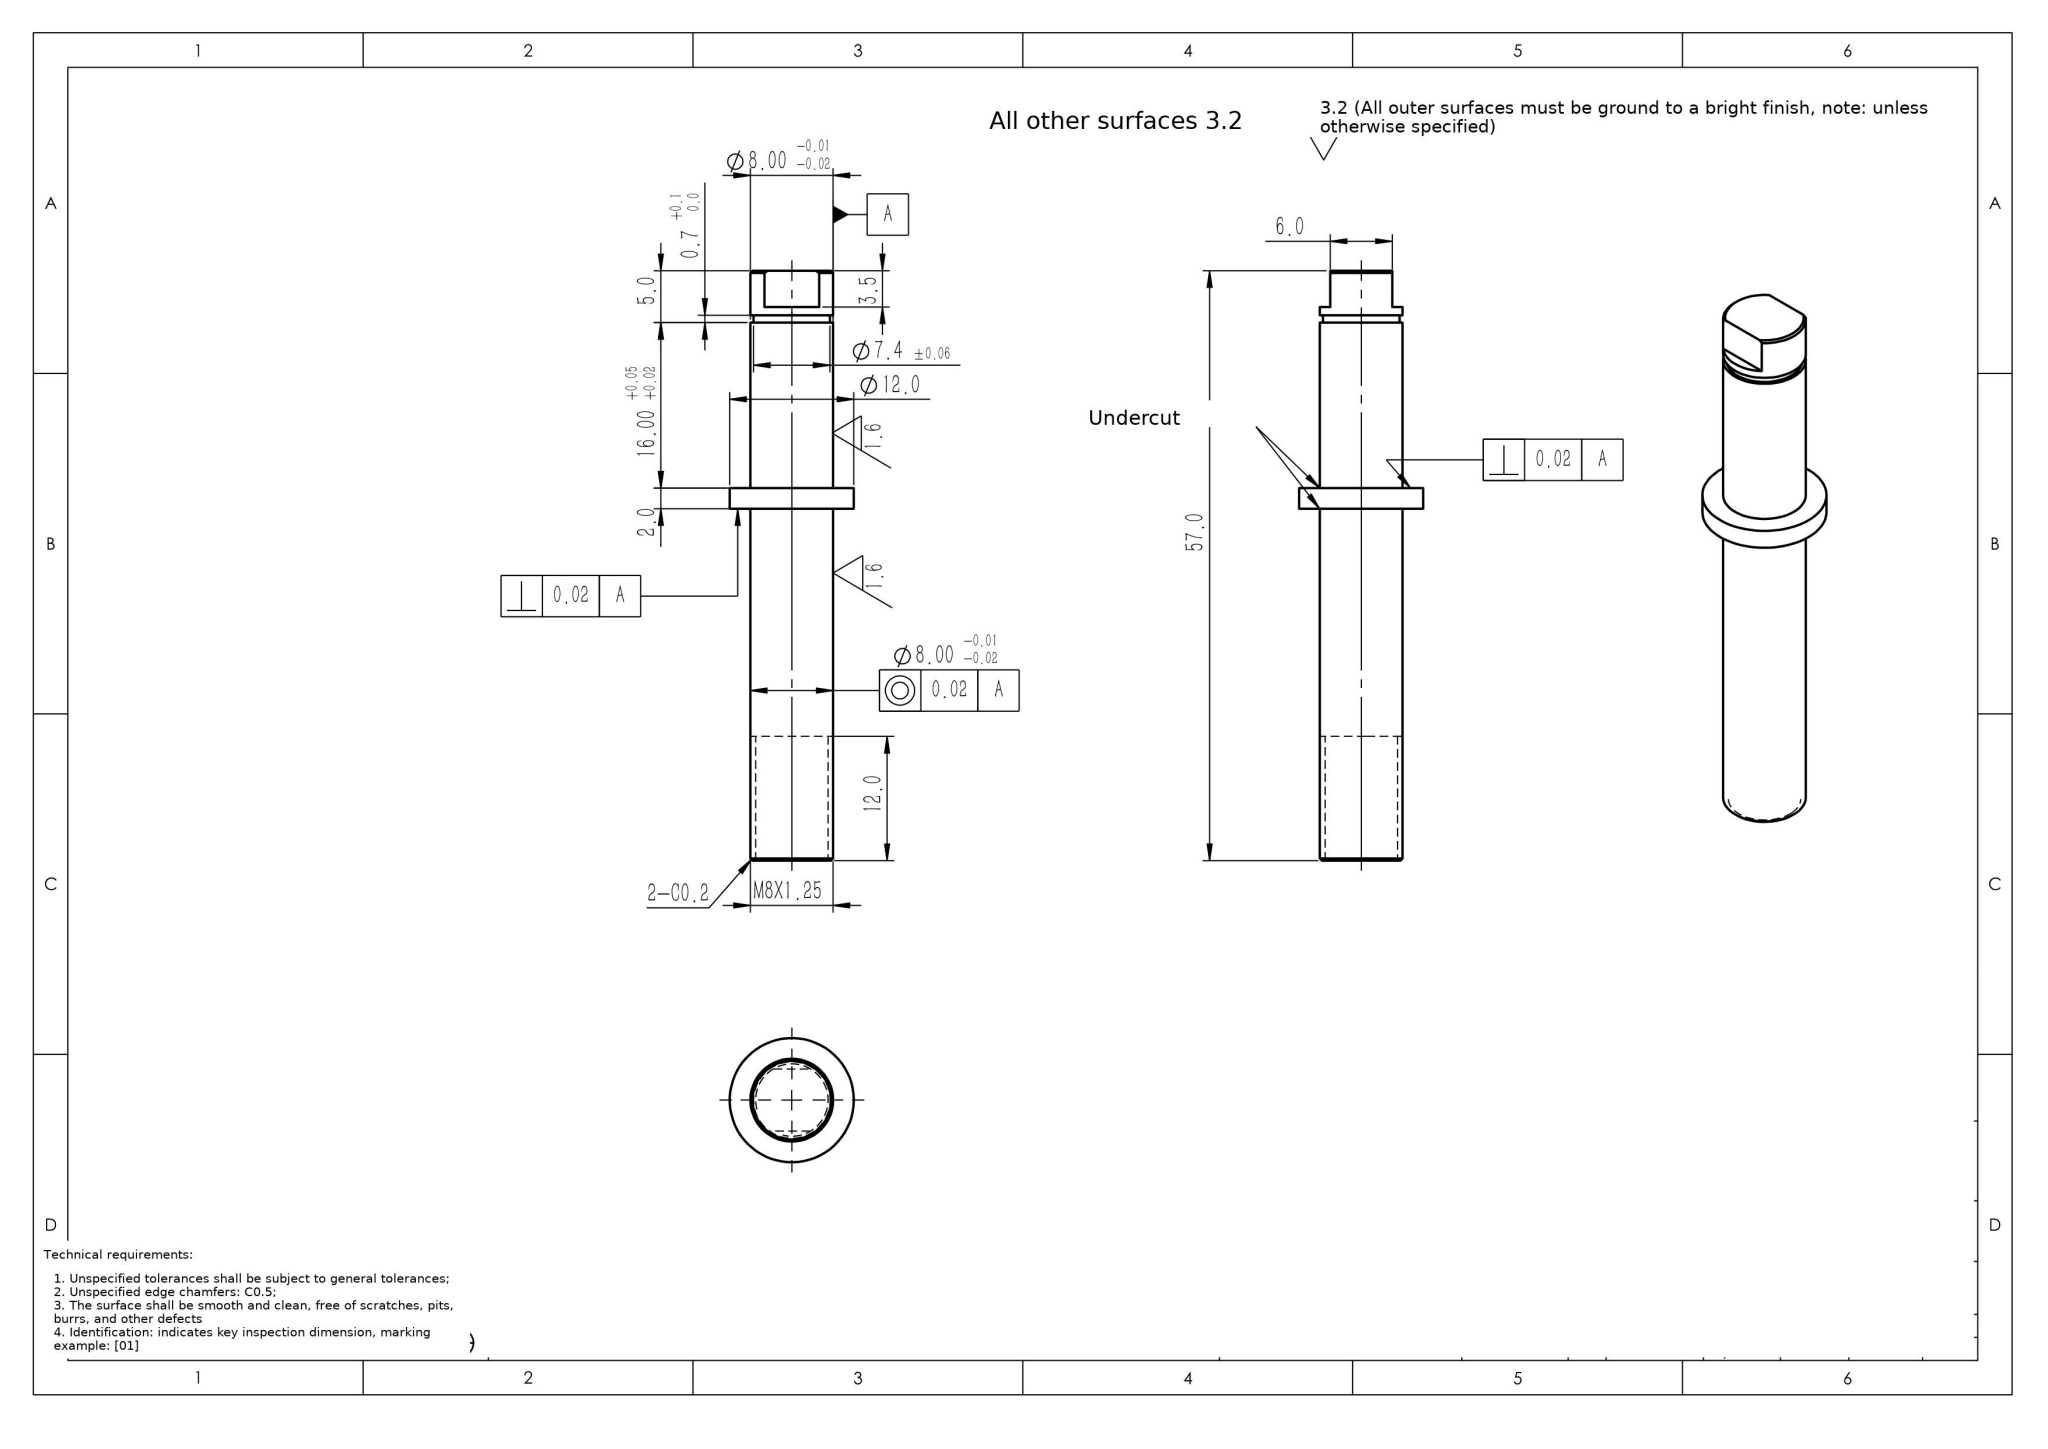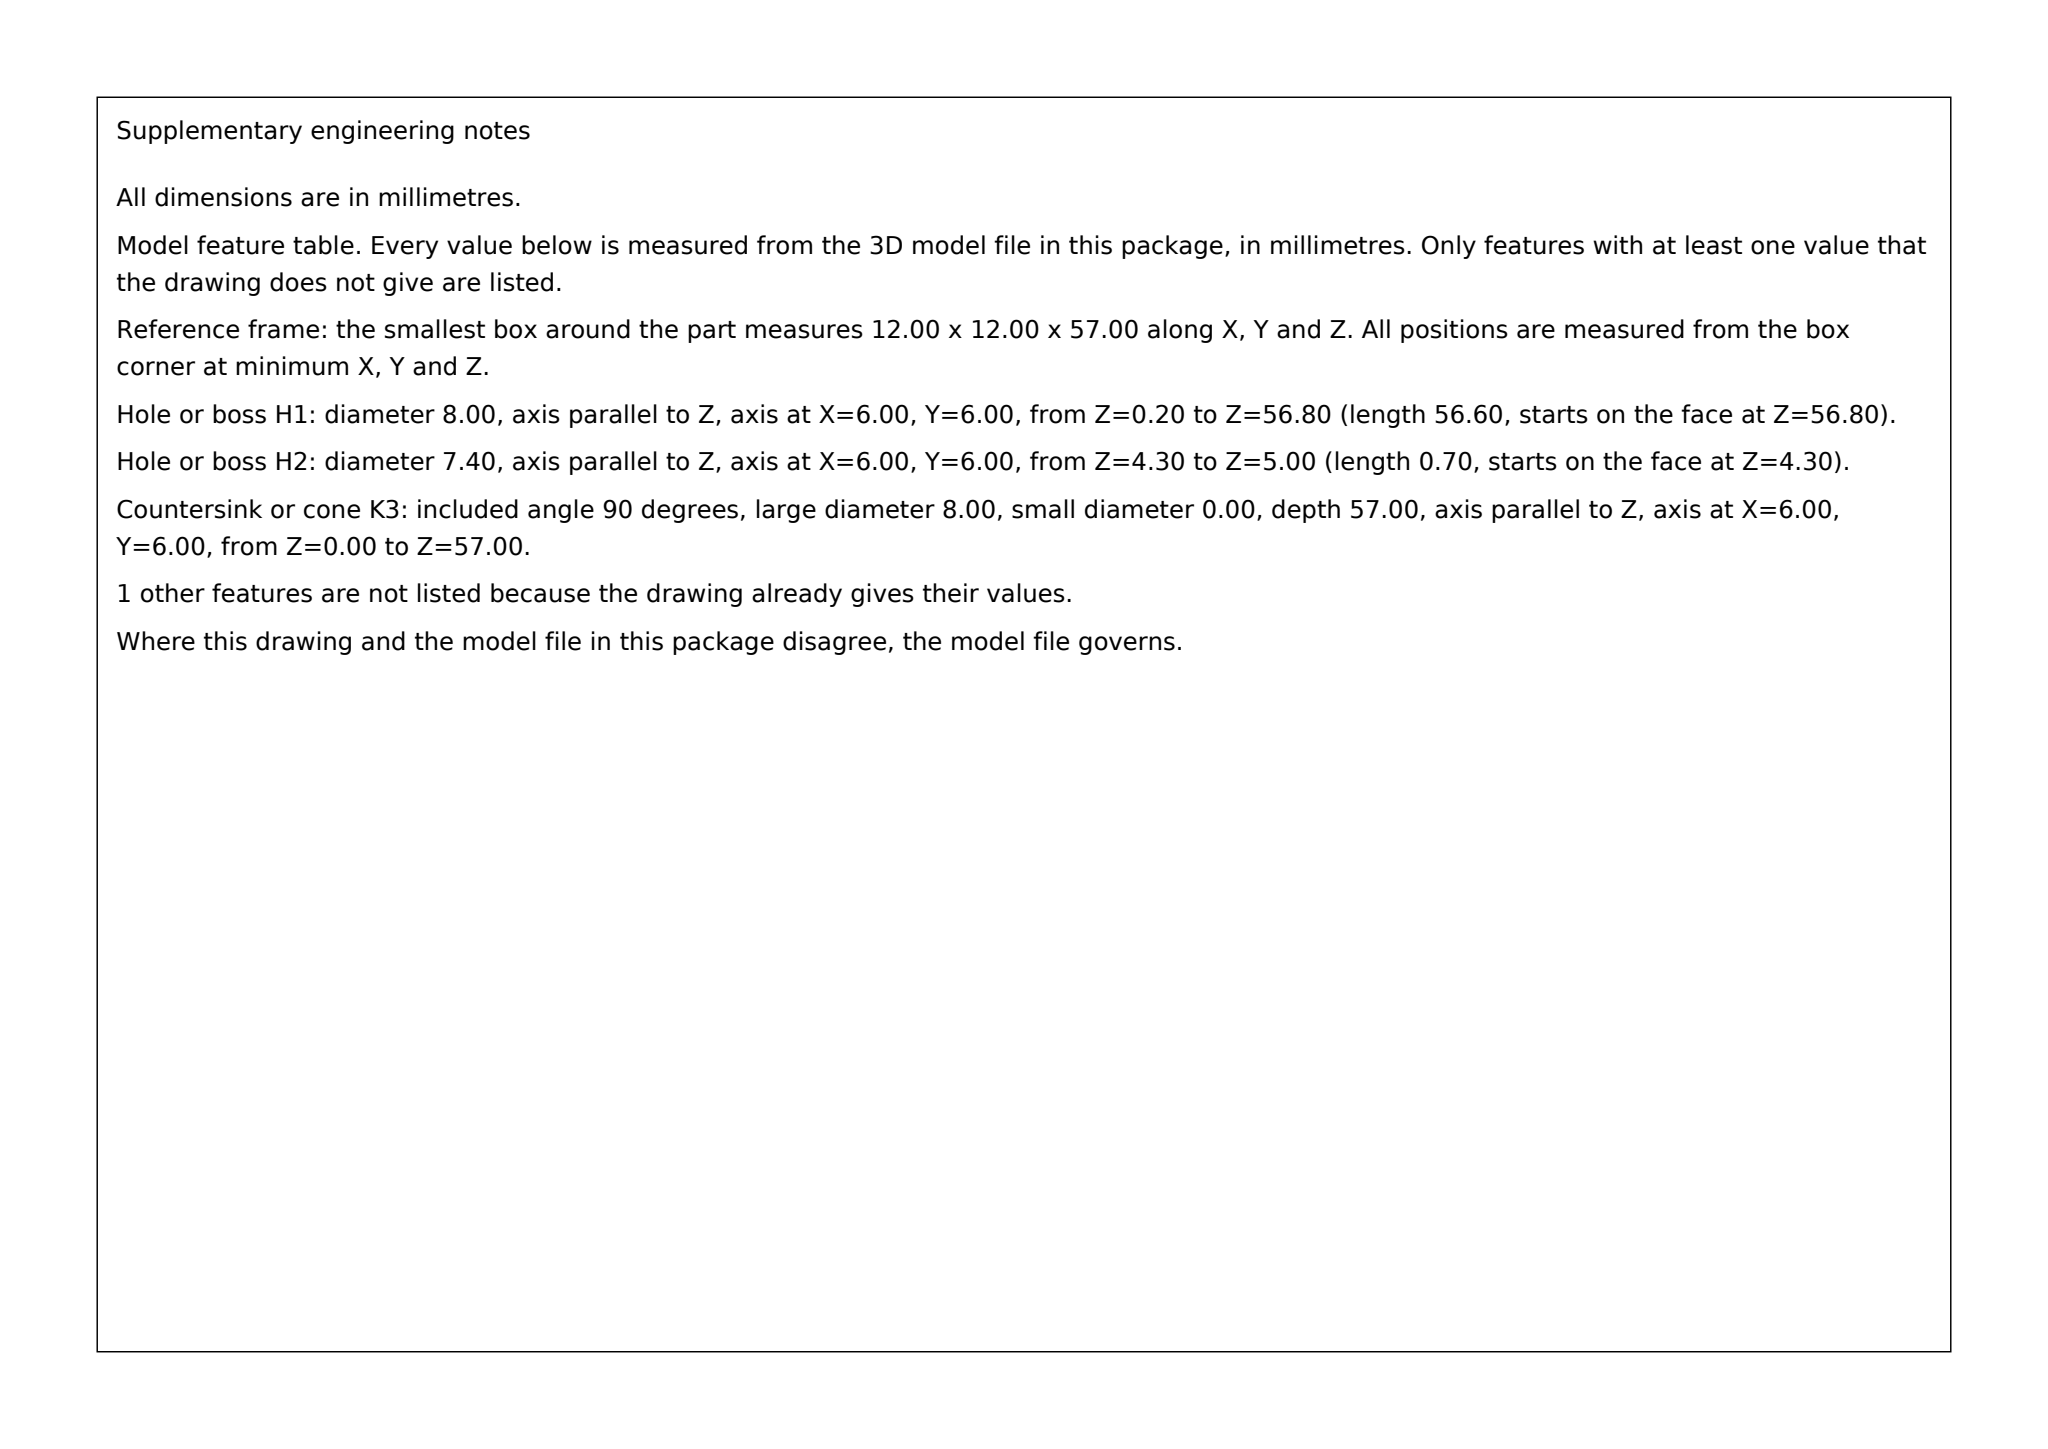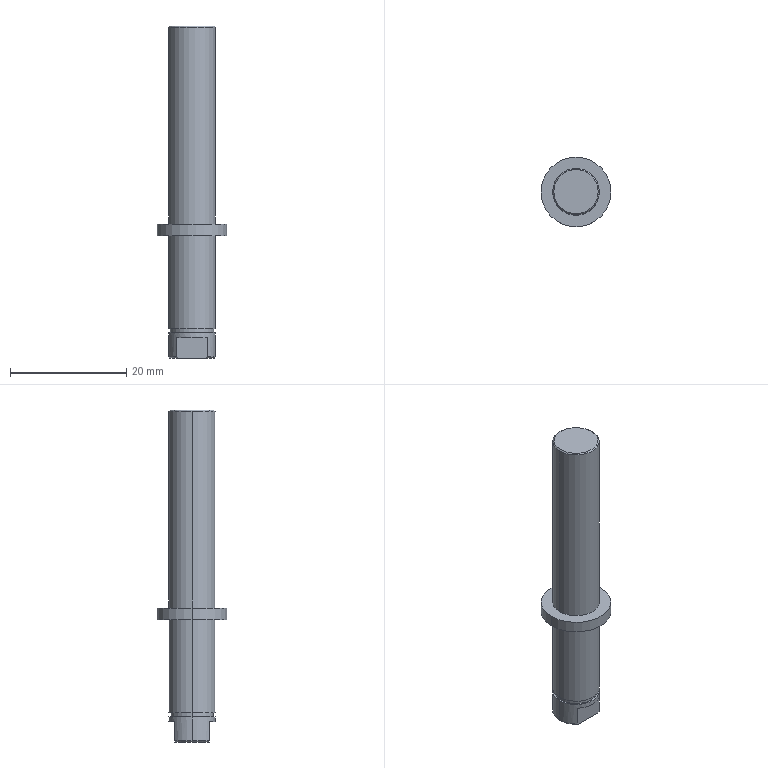Part | SolidWorks | mm | 1 solid | 25 faces | box 12 x 12 x 57 mm | volume 2960 mm3 | cylinder 10 | plane 10 | cone 5 | commonest cylinder face diameters 8 x6 7.4 x2 12 x2
build123d program:
from build123d import *

# Parameters (mm, degrees)
SKETCH1_R           = 6
BOSS_EXTRUDE1_DEPTH = 2
SKETCH2_R           = 4
BOSS_EXTRUDE2_DEPTH = 36
BOSS_EXTRUDE4_START = 21
SKETCH3_R           = 4
BOSS_EXTRUDE4_DEPTH = 21
SKETCH5_W           = 0.3
SKETCH5_H           = 0.7
CUT_EXTRUDE1_DEPTH  = 3.5
CHAMFER1_SIZE       = 0.2


with BuildPart() as part:
    # Sketch1 → Boss-Extrude1 (new body)
    with BuildSketch(Plane.XY):
        Circle(SKETCH1_R)
    extrude(amount=BOSS_EXTRUDE1_DEPTH)

    # Sketch2 → Boss-Extrude2 (add)
    with BuildSketch(Plane.XY):
        Circle(SKETCH2_R)
    extrude(amount=BOSS_EXTRUDE2_DEPTH)

    # Sketch3 → Boss-Extrude4 (add)
    with BuildSketch(Plane(origin=(0, 0, 0), x_dir=(-1, 0, 0), z_dir=(0, 0, -1)).offset(BOSS_EXTRUDE4_START)):
        with Locations(Location((0, 0, 0), (0, 0, 180))):
            Circle(SKETCH3_R)
    extrude(amount=-BOSS_EXTRUDE4_DEPTH)

    # Sketch5 → Cut-Revolve1 (revolve, cut)
    with BuildSketch(Plane(origin=(0, 0, 0), x_dir=(1, 0, 0), z_dir=(0, 1, 0))):
        with Locations((3.85, 16.35)):
            Rectangle(SKETCH5_W, SKETCH5_H)
    revolve(axis=Axis((0, 0, 0), (0, 0, -1)), mode=Mode.SUBTRACT)

    # Sketch6 → Cut-Extrude1 (cut)
    with BuildSketch(Plane(origin=(0, 0, -21), x_dir=(-1, 0, 0), z_dir=(0, 0, -1))):
        with BuildLine():
            Line((-2.646, 3), (2.646, 3))
            ThreePointArc((2.646, 3), (0, 4), (-2.646, 3))
        make_face()
        with BuildLine():
            Line((2.646, -3), (-2.646, -3))
            ThreePointArc((-2.646, -3), (0, -4), (2.646, -3))
        make_face()
    extrude(amount=-CUT_EXTRUDE1_DEPTH, mode=Mode.SUBTRACT)

    # Chamfer1
    chamfer1_edges = [part.edges().sort_by_distance(p)[0] for p in [
        (-4, 0, -21),
        (3.646, -1.646, -21),
        (-4, 0, 36),
    ]]
    chamfer(chamfer1_edges, length=CHAMFER1_SIZE)


solid = part.part
STEP:
#1=CARTESIAN_POINT('',(3.8,0.,36.));
#2=VERTEX_POINT('',#1);
#3=CARTESIAN_POINT('',(-3.8,0.,36.));
#4=VERTEX_POINT('',#3);
#5=CARTESIAN_POINT('',(0.,0.,36.));
#6=DIRECTION('',(0.,0.,1.));
#7=DIRECTION('',(1.,0.,0.));
#8=AXIS2_PLACEMENT_3D('',#5,#6,#7);
#9=CIRCLE('',#8,3.8);
#10=EDGE_CURVE('',#2,#4,#9,.T.);
#11=ORIENTED_EDGE('',*,*,#10,.F.);
#12=CARTESIAN_POINT('',(4.,0.,35.8));
#13=VERTEX_POINT('',#12);
#14=CARTESIAN_POINT('',(3.8,0.,36.));
#15=DIRECTION('',(0.7071,0.,-0.7071));
#16=VECTOR('',#15,1000.);
#17=LINE('',#14,#16);
#18=EDGE_CURVE('',#2,#13,#17,.T.);
#19=ORIENTED_EDGE('',*,*,#18,.T.);
#20=CARTESIAN_POINT('',(-4.,0.,35.8));
#21=VERTEX_POINT('',#20);
#22=CARTESIAN_POINT('',(0.,0.,35.8));
#23=DIRECTION('',(0.,0.,-1.));
#24=DIRECTION('',(1.,0.,0.));
#25=AXIS2_PLACEMENT_3D('',#22,#23,#24);
#26=CIRCLE('',#25,4.);
#27=EDGE_CURVE('',#21,#13,#26,.T.);
#28=ORIENTED_EDGE('',*,*,#27,.F.);
#29=CARTESIAN_POINT('',(-3.8,0.,36.));
#30=DIRECTION('',(-0.7071,0.,-0.7071));
#31=VECTOR('',#30,1000.);
#32=LINE('',#29,#31);
#33=EDGE_CURVE('',#4,#21,#32,.T.);
#34=ORIENTED_EDGE('',*,*,#33,.F.);
#35=EDGE_LOOP('',(#11,#19,#28,#34));
#36=FACE_OUTER_BOUND('',#35,.T.);
#37=CARTESIAN_POINT('',(0.,0.,36.));
#38=DIRECTION('',(0.,0.,-1.));
#39=DIRECTION('',(-1.,0.,0.));
#40=AXIS2_PLACEMENT_3D('',#37,#38,#39);
#41=CONICAL_SURFACE('',#40,3.8,0.7854);
#42=ADVANCED_FACE('',(#36),#41,.T.);
#43=CARTESIAN_POINT('',(3.8,0.,-21.));
#44=VERTEX_POINT('',#43);
#45=CARTESIAN_POINT('',(2.332,-3.,-21.));
#46=VERTEX_POINT('',#45);
#47=CARTESIAN_POINT('',(0.,0.,-21.));
#48=DIRECTION('',(0.,0.,-1.));
#49=DIRECTION('',(-1.,0.,0.));
#50=AXIS2_PLACEMENT_3D('',#47,#48,#49);
#51=CIRCLE('',#50,3.8);
#52=EDGE_CURVE('',#44,#46,#51,.T.);
#53=ORIENTED_EDGE('',*,*,#52,.F.);
#54=CARTESIAN_POINT('',(4.,0.,-20.8));
#55=VERTEX_POINT('',#54);
#56=CARTESIAN_POINT('',(3.8,0.,-21.));
#57=DIRECTION('',(0.7071,0.,0.7071));
#58=VECTOR('',#57,1000.);
#59=LINE('',#56,#58);
#60=EDGE_CURVE('',#44,#55,#59,.T.);
#61=ORIENTED_EDGE('',*,*,#60,.T.);
#62=CARTESIAN_POINT('',(2.646,-3.,-20.8));
#63=VERTEX_POINT('',#62);
#64=CARTESIAN_POINT('',(0.,0.,-20.8));
#65=DIRECTION('',(0.,0.,1.));
#66=DIRECTION('',(-1.,0.,0.));
#67=AXIS2_PLACEMENT_3D('',#64,#65,#66);
#68=CIRCLE('',#67,4.);
#69=EDGE_CURVE('',#63,#55,#68,.T.);
#70=ORIENTED_EDGE('',*,*,#69,.F.);
#71=CARTESIAN_POINT('',(2.332,-3.,-21.));
#72=CARTESIAN_POINT('',(2.438,-3.,-20.935));
#73=CARTESIAN_POINT('',(2.542,-3.,-20.868));
#74=CARTESIAN_POINT('',(2.646,-3.,-20.8));
#75=B_SPLINE_CURVE_WITH_KNOTS('',3,(#71,#72,#73,#74),.UNSPECIFIED.,.F.,.F.,(4,4),(0.,0.0003718),.UNSPECIFIED.);
#76=EDGE_CURVE('',#46,#63,#75,.T.);
#77=ORIENTED_EDGE('',*,*,#76,.F.);
#78=EDGE_LOOP('',(#53,#61,#70,#77));
#79=FACE_OUTER_BOUND('',#78,.T.);
#80=CARTESIAN_POINT('',(0.,0.,-21.));
#81=DIRECTION('',(0.,0.,1.));
#82=DIRECTION('',(1.,0.,0.));
#83=AXIS2_PLACEMENT_3D('',#80,#81,#82);
#84=CONICAL_SURFACE('',#83,3.8,0.7854);
#85=ADVANCED_FACE('',(#79),#84,.T.);
#86=CARTESIAN_POINT('',(-2.646,3.,-20.8));
#87=VERTEX_POINT('',#86);
#88=CARTESIAN_POINT('',(-4.,0.,-20.8));
#89=VERTEX_POINT('',#88);
#90=CARTESIAN_POINT('',(0.,0.,-20.8));
#91=DIRECTION('',(0.,0.,1.));
#92=DIRECTION('',(-1.,-0.,0.));
#93=AXIS2_PLACEMENT_3D('',#90,#91,#92);
#94=CIRCLE('',#93,4.);
#95=EDGE_CURVE('',#87,#89,#94,.T.);
#96=ORIENTED_EDGE('',*,*,#95,.T.);
#97=CARTESIAN_POINT('',(-4.,0.,-16.7));
#98=VERTEX_POINT('',#97);
#99=CARTESIAN_POINT('',(-4.,0.,-21.));
#100=DIRECTION('',(0.,0.,1.));
#101=VECTOR('',#100,1000.);
#102=LINE('',#99,#101);
#103=EDGE_CURVE('',#89,#98,#102,.T.);
#104=ORIENTED_EDGE('',*,*,#103,.T.);
#105=CARTESIAN_POINT('',(4.,0.,-16.7));
#106=VERTEX_POINT('',#105);
#107=CARTESIAN_POINT('',(0.,0.,-16.7));
#108=DIRECTION('',(0.,0.,1.));
#109=DIRECTION('',(1.,0.,0.));
#110=AXIS2_PLACEMENT_3D('',#107,#108,#109);
#111=CIRCLE('',#110,4.);
#112=EDGE_CURVE('',#106,#98,#111,.T.);
#113=ORIENTED_EDGE('',*,*,#112,.F.);
#114=CARTESIAN_POINT('',(4.,0.,-21.));
#115=DIRECTION('',(0.,0.,1.));
#116=VECTOR('',#115,1000.);
#117=LINE('',#114,#116);
#118=EDGE_CURVE('',#55,#106,#117,.T.);
#119=ORIENTED_EDGE('',*,*,#118,.F.);
#120=CARTESIAN_POINT('',(2.646,3.,-20.8));
#121=VERTEX_POINT('',#120);
#122=CARTESIAN_POINT('',(0.,0.,-20.8));
#123=DIRECTION('',(0.,0.,1.));
#124=DIRECTION('',(-1.,0.,0.));
#125=AXIS2_PLACEMENT_3D('',#122,#123,#124);
#126=CIRCLE('',#125,4.);
#127=EDGE_CURVE('',#55,#121,#126,.T.);
#128=ORIENTED_EDGE('',*,*,#127,.T.);
#129=CARTESIAN_POINT('',(2.646,3.,-17.5));
#130=VERTEX_POINT('',#129);
#131=CARTESIAN_POINT('',(2.646,3.,-17.5));
#132=DIRECTION('',(0.,0.,-1.));
#133=VECTOR('',#132,1000.);
#134=LINE('',#131,#133);
#135=EDGE_CURVE('',#130,#121,#134,.T.);
#136=ORIENTED_EDGE('',*,*,#135,.F.);
#137=CARTESIAN_POINT('',(-2.646,3.,-17.5));
#138=VERTEX_POINT('',#137);
#139=CARTESIAN_POINT('',(0.,0.,-17.5));
#140=DIRECTION('',(0.,0.,-1.));
#141=DIRECTION('',(-1.,0.,0.));
#142=AXIS2_PLACEMENT_3D('',#139,#140,#141);
#143=CIRCLE('',#142,4.);
#144=EDGE_CURVE('',#138,#130,#143,.T.);
#145=ORIENTED_EDGE('',*,*,#144,.F.);
#146=CARTESIAN_POINT('',(-2.646,3.,-17.5));
#147=DIRECTION('',(0.,0.,-1.));
#148=VECTOR('',#147,1000.);
#149=LINE('',#146,#148);
#150=EDGE_CURVE('',#138,#87,#149,.T.);
#151=ORIENTED_EDGE('',*,*,#150,.T.);
#152=EDGE_LOOP('',(#96,#104,#113,#119,#128,#136,#145,#151));
#153=FACE_OUTER_BOUND('',#152,.T.);
#154=CARTESIAN_POINT('',(0.,0.,-21.));
#155=DIRECTION('',(0.,0.,1.));
#156=DIRECTION('',(1.,0.,0.));
#157=AXIS2_PLACEMENT_3D('',#154,#155,#156);
#158=CYLINDRICAL_SURFACE('',#157,4.);
#159=ADVANCED_FACE('',(#153),#158,.T.);
#160=CARTESIAN_POINT('',(3.7,0.,-16.7));
#161=VERTEX_POINT('',#160);
#162=CARTESIAN_POINT('',(-3.7,0.,-16.7));
#163=VERTEX_POINT('',#162);
#164=CARTESIAN_POINT('',(0.,0.,-16.7));
#165=DIRECTION('',(0.,0.,1.));
#166=DIRECTION('',(1.,0.,0.));
#167=AXIS2_PLACEMENT_3D('',#164,#165,#166);
#168=CIRCLE('',#167,3.7);
#169=EDGE_CURVE('',#161,#163,#168,.T.);
#170=ORIENTED_EDGE('',*,*,#169,.T.);
#171=CARTESIAN_POINT('',(-3.7,0.,-16.));
#172=VERTEX_POINT('',#171);
#173=CARTESIAN_POINT('',(-3.7,0.,0.));
#174=DIRECTION('',(0.,0.,1.));
#175=VECTOR('',#174,1000.);
#176=LINE('',#173,#175);
#177=EDGE_CURVE('',#163,#172,#176,.T.);
#178=ORIENTED_EDGE('',*,*,#177,.T.);
#179=CARTESIAN_POINT('',(3.7,0.,-16.));
#180=VERTEX_POINT('',#179);
#181=CARTESIAN_POINT('',(0.,0.,-16.));
#182=DIRECTION('',(0.,0.,1.));
#183=DIRECTION('',(1.,0.,0.));
#184=AXIS2_PLACEMENT_3D('',#181,#182,#183);
#185=CIRCLE('',#184,3.7);
#186=EDGE_CURVE('',#180,#172,#185,.T.);
#187=ORIENTED_EDGE('',*,*,#186,.F.);
#188=CARTESIAN_POINT('',(3.7,0.,0.));
#189=DIRECTION('',(0.,0.,1.));
#190=VECTOR('',#189,1000.);
#191=LINE('',#188,#190);
#192=EDGE_CURVE('',#161,#180,#191,.T.);
#193=ORIENTED_EDGE('',*,*,#192,.F.);
#194=EDGE_LOOP('',(#170,#178,#187,#193));
#195=FACE_OUTER_BOUND('',#194,.T.);
#196=CARTESIAN_POINT('',(0.,0.,0.));
#197=DIRECTION('',(0.,0.,1.));
#198=DIRECTION('',(1.,0.,0.));
#199=AXIS2_PLACEMENT_3D('',#196,#197,#198);
#200=CYLINDRICAL_SURFACE('',#199,3.7);
#201=ADVANCED_FACE('',(#195),#200,.T.);
#202=ORIENTED_EDGE('',*,*,#27,.T.);
#203=CARTESIAN_POINT('',(4.,0.,2.));
#204=VERTEX_POINT('',#203);
#205=CARTESIAN_POINT('',(4.,0.,36.));
#206=DIRECTION('',(0.,0.,-1.));
#207=VECTOR('',#206,1000.);
#208=LINE('',#205,#207);
#209=EDGE_CURVE('',#13,#204,#208,.T.);
#210=ORIENTED_EDGE('',*,*,#209,.T.);
#211=CARTESIAN_POINT('',(-4.,0.,2.));
#212=VERTEX_POINT('',#211);
#213=CARTESIAN_POINT('',(0.,0.,2.));
#214=DIRECTION('',(0.,0.,-1.));
#215=DIRECTION('',(1.,0.,0.));
#216=AXIS2_PLACEMENT_3D('',#213,#214,#215);
#217=CIRCLE('',#216,4.);
#218=EDGE_CURVE('',#212,#204,#217,.T.);
#219=ORIENTED_EDGE('',*,*,#218,.F.);
#220=CARTESIAN_POINT('',(-4.,0.,36.));
#221=DIRECTION('',(0.,0.,-1.));
#222=VECTOR('',#221,1000.);
#223=LINE('',#220,#222);
#224=EDGE_CURVE('',#21,#212,#223,.T.);
#225=ORIENTED_EDGE('',*,*,#224,.F.);
#226=EDGE_LOOP('',(#202,#210,#219,#225));
#227=FACE_OUTER_BOUND('',#226,.T.);
#228=CARTESIAN_POINT('',(0.,0.,36.));
#229=DIRECTION('',(0.,0.,-1.));
#230=DIRECTION('',(-1.,0.,0.));
#231=AXIS2_PLACEMENT_3D('',#228,#229,#230);
#232=CYLINDRICAL_SURFACE('',#231,4.);
#233=ADVANCED_FACE('',(#227),#232,.T.);
#234=CARTESIAN_POINT('',(6.,0.,2.));
#235=VERTEX_POINT('',#234);
#236=CARTESIAN_POINT('',(-6.,0.,2.));
#237=VERTEX_POINT('',#236);
#238=CARTESIAN_POINT('',(0.,0.,2.));
#239=DIRECTION('',(0.,0.,1.));
#240=DIRECTION('',(1.,0.,0.));
#241=AXIS2_PLACEMENT_3D('',#238,#239,#240);
#242=CIRCLE('',#241,6.);
#243=EDGE_CURVE('',#235,#237,#242,.T.);
#244=ORIENTED_EDGE('',*,*,#243,.F.);
#245=CARTESIAN_POINT('',(6.,0.,0.));
#246=VERTEX_POINT('',#245);
#247=CARTESIAN_POINT('',(6.,0.,2.));
#248=DIRECTION('',(0.,0.,-1.));
#249=VECTOR('',#248,1000.);
#250=LINE('',#247,#249);
#251=EDGE_CURVE('',#235,#246,#250,.T.);
#252=ORIENTED_EDGE('',*,*,#251,.T.);
#253=CARTESIAN_POINT('',(-6.,0.,0.));
#254=VERTEX_POINT('',#253);
#255=CARTESIAN_POINT('',(0.,0.,0.));
#256=DIRECTION('',(0.,0.,1.));
#257=DIRECTION('',(1.,0.,0.));
#258=AXIS2_PLACEMENT_3D('',#255,#256,#257);
#259=CIRCLE('',#258,6.);
#260=EDGE_CURVE('',#246,#254,#259,.T.);
#261=ORIENTED_EDGE('',*,*,#260,.T.);
#262=CARTESIAN_POINT('',(-6.,0.,2.));
#263=DIRECTION('',(0.,0.,-1.));
#264=VECTOR('',#263,1000.);
#265=LINE('',#262,#264);
#266=EDGE_CURVE('',#237,#254,#265,.T.);
#267=ORIENTED_EDGE('',*,*,#266,.F.);
#268=EDGE_LOOP('',(#244,#252,#261,#267));
#269=FACE_OUTER_BOUND('',#268,.T.);
#270=CARTESIAN_POINT('',(0.,0.,2.));
#271=DIRECTION('',(0.,0.,-1.));
#272=DIRECTION('',(-1.,0.,0.));
#273=AXIS2_PLACEMENT_3D('',#270,#271,#272);
#274=CYLINDRICAL_SURFACE('',#273,6.);
#275=ADVANCED_FACE('',(#269),#274,.T.);
#276=CARTESIAN_POINT('',(4.,0.,-16.));
#277=VERTEX_POINT('',#276);
#278=CARTESIAN_POINT('',(-4.,0.,-16.));
#279=VERTEX_POINT('',#278);
#280=CARTESIAN_POINT('',(0.,0.,-16.));
#281=DIRECTION('',(0.,0.,1.));
#282=DIRECTION('',(1.,0.,0.));
#283=AXIS2_PLACEMENT_3D('',#280,#281,#282);
#284=CIRCLE('',#283,4.);
#285=EDGE_CURVE('',#277,#279,#284,.T.);
#286=ORIENTED_EDGE('',*,*,#285,.T.);
#287=CARTESIAN_POINT('',(-4.,0.,0.));
#288=VERTEX_POINT('',#287);
#289=CARTESIAN_POINT('',(-4.,0.,-21.));
#290=DIRECTION('',(0.,0.,1.));
#291=VECTOR('',#290,1000.);
#292=LINE('',#289,#291);
#293=EDGE_CURVE('',#279,#288,#292,.T.);
#294=ORIENTED_EDGE('',*,*,#293,.T.);
#295=CARTESIAN_POINT('',(4.,0.,0.));
#296=VERTEX_POINT('',#295);
#297=CARTESIAN_POINT('',(0.,0.,0.));
#298=DIRECTION('',(0.,0.,-1.));
#299=DIRECTION('',(1.,0.,0.));
#300=AXIS2_PLACEMENT_3D('',#297,#298,#299);
#301=CIRCLE('',#300,4.);
#302=EDGE_CURVE('',#288,#296,#301,.T.);
#303=ORIENTED_EDGE('',*,*,#302,.T.);
#304=CARTESIAN_POINT('',(4.,0.,-21.));
#305=DIRECTION('',(0.,0.,1.));
#306=VECTOR('',#305,1000.);
#307=LINE('',#304,#306);
#308=EDGE_CURVE('',#277,#296,#307,.T.);
#309=ORIENTED_EDGE('',*,*,#308,.F.);
#310=EDGE_LOOP('',(#286,#294,#303,#309));
#311=FACE_OUTER_BOUND('',#310,.T.);
#312=CARTESIAN_POINT('',(0.,0.,-21.));
#313=DIRECTION('',(0.,0.,1.));
#314=DIRECTION('',(1.,0.,0.));
#315=AXIS2_PLACEMENT_3D('',#312,#313,#314);
#316=CYLINDRICAL_SURFACE('',#315,4.);
#317=ADVANCED_FACE('',(#311),#316,.T.);
#318=ORIENTED_EDGE('',*,*,#293,.F.);
#319=CARTESIAN_POINT('',(0.,0.,-16.));
#320=DIRECTION('',(0.,0.,1.));
#321=DIRECTION('',(1.,0.,0.));
#322=AXIS2_PLACEMENT_3D('',#319,#320,#321);
#323=CIRCLE('',#322,4.);
#324=EDGE_CURVE('',#279,#277,#323,.T.);
#325=ORIENTED_EDGE('',*,*,#324,.T.);
#326=ORIENTED_EDGE('',*,*,#308,.T.);
#327=CARTESIAN_POINT('',(0.,0.,0.));
#328=DIRECTION('',(0.,0.,-1.));
#329=DIRECTION('',(1.,0.,0.));
#330=AXIS2_PLACEMENT_3D('',#327,#328,#329);
#331=CIRCLE('',#330,4.);
#332=EDGE_CURVE('',#296,#288,#331,.T.);
#333=ORIENTED_EDGE('',*,*,#332,.T.);
#334=EDGE_LOOP('',(#318,#325,#326,#333));
#335=FACE_OUTER_BOUND('',#334,.T.);
#336=CARTESIAN_POINT('',(0.,0.,-21.));
#337=DIRECTION('',(0.,0.,1.));
#338=DIRECTION('',(1.,0.,0.));
#339=AXIS2_PLACEMENT_3D('',#336,#337,#338);
#340=CYLINDRICAL_SURFACE('',#339,4.);
#341=ADVANCED_FACE('',(#335),#340,.T.);
#342=CARTESIAN_POINT('',(0.,0.,0.));
#343=DIRECTION('',(0.,0.,1.));
#344=DIRECTION('',(1.,0.,0.));
#345=AXIS2_PLACEMENT_3D('',#342,#343,#344);
#346=CIRCLE('',#345,6.);
#347=EDGE_CURVE('',#254,#246,#346,.T.);
#348=ORIENTED_EDGE('',*,*,#347,.F.);
#349=ORIENTED_EDGE('',*,*,#260,.F.);
#350=EDGE_LOOP('',(#348,#349));
#351=FACE_OUTER_BOUND('',#350,.T.);
#352=ORIENTED_EDGE('',*,*,#332,.F.);
#353=ORIENTED_EDGE('',*,*,#302,.F.);
#354=EDGE_LOOP('',(#352,#353));
#355=FACE_BOUND('',#354,.T.);
#356=CARTESIAN_POINT('',(0.,0.,0.));
#357=DIRECTION('',(0.,0.,1.));
#358=DIRECTION('',(1.,0.,0.));
#359=AXIS2_PLACEMENT_3D('',#356,#357,#358);
#360=PLANE('',#359);
#361=ADVANCED_FACE('',(#351,#355),#360,.F.);
#362=CARTESIAN_POINT('',(0.,0.,2.));
#363=DIRECTION('',(0.,0.,1.));
#364=DIRECTION('',(1.,0.,0.));
#365=AXIS2_PLACEMENT_3D('',#362,#363,#364);
#366=CIRCLE('',#365,6.);
#367=EDGE_CURVE('',#237,#235,#366,.T.);
#368=ORIENTED_EDGE('',*,*,#367,.T.);
#369=ORIENTED_EDGE('',*,*,#243,.T.);
#370=EDGE_LOOP('',(#368,#369));
#371=FACE_OUTER_BOUND('',#370,.T.);
#372=ORIENTED_EDGE('',*,*,#218,.T.);
#373=CARTESIAN_POINT('',(0.,0.,2.));
#374=DIRECTION('',(0.,0.,-1.));
#375=DIRECTION('',(1.,0.,0.));
#376=AXIS2_PLACEMENT_3D('',#373,#374,#375);
#377=CIRCLE('',#376,4.);
#378=EDGE_CURVE('',#204,#212,#377,.T.);
#379=ORIENTED_EDGE('',*,*,#378,.T.);
#380=EDGE_LOOP('',(#372,#379));
#381=FACE_BOUND('',#380,.T.);
#382=CARTESIAN_POINT('',(0.,0.,2.));
#383=DIRECTION('',(0.,0.,1.));
#384=DIRECTION('',(1.,0.,0.));
#385=AXIS2_PLACEMENT_3D('',#382,#383,#384);
#386=PLANE('',#385);
#387=ADVANCED_FACE('',(#371,#381),#386,.T.);
#388=ORIENTED_EDGE('',*,*,#251,.F.);
#389=ORIENTED_EDGE('',*,*,#367,.F.);
#390=ORIENTED_EDGE('',*,*,#266,.T.);
#391=ORIENTED_EDGE('',*,*,#347,.T.);
#392=EDGE_LOOP('',(#388,#389,#390,#391));
#393=FACE_OUTER_BOUND('',#392,.T.);
#394=CARTESIAN_POINT('',(0.,0.,2.));
#395=DIRECTION('',(0.,0.,-1.));
#396=DIRECTION('',(-1.,0.,0.));
#397=AXIS2_PLACEMENT_3D('',#394,#395,#396);
#398=CYLINDRICAL_SURFACE('',#397,6.);
#399=ADVANCED_FACE('',(#393),#398,.T.);
#400=ORIENTED_EDGE('',*,*,#209,.F.);
#401=CARTESIAN_POINT('',(0.,0.,35.8));
#402=DIRECTION('',(0.,0.,-1.));
#403=DIRECTION('',(1.,0.,0.));
#404=AXIS2_PLACEMENT_3D('',#401,#402,#403);
#405=CIRCLE('',#404,4.);
#406=EDGE_CURVE('',#13,#21,#405,.T.);
#407=ORIENTED_EDGE('',*,*,#406,.T.);
#408=ORIENTED_EDGE('',*,*,#224,.T.);
#409=ORIENTED_EDGE('',*,*,#378,.F.);
#410=EDGE_LOOP('',(#400,#407,#408,#409));
#411=FACE_OUTER_BOUND('',#410,.T.);
#412=CARTESIAN_POINT('',(0.,0.,36.));
#413=DIRECTION('',(0.,0.,-1.));
#414=DIRECTION('',(-1.,0.,0.));
#415=AXIS2_PLACEMENT_3D('',#412,#413,#414);
#416=CYLINDRICAL_SURFACE('',#415,4.);
#417=ADVANCED_FACE('',(#411),#416,.T.);
#418=CARTESIAN_POINT('',(0.,0.,36.));
#419=DIRECTION('',(0.,0.,1.));
#420=DIRECTION('',(1.,0.,0.));
#421=AXIS2_PLACEMENT_3D('',#418,#419,#420);
#422=CIRCLE('',#421,3.8);
#423=EDGE_CURVE('',#4,#2,#422,.T.);
#424=ORIENTED_EDGE('',*,*,#423,.T.);
#425=ORIENTED_EDGE('',*,*,#10,.T.);
#426=EDGE_LOOP('',(#424,#425));
#427=FACE_OUTER_BOUND('',#426,.T.);
#428=CARTESIAN_POINT('',(0.,0.,36.));
#429=DIRECTION('',(0.,0.,1.));
#430=DIRECTION('',(1.,0.,0.));
#431=AXIS2_PLACEMENT_3D('',#428,#429,#430);
#432=PLANE('',#431);
#433=ADVANCED_FACE('',(#427),#432,.T.);
#434=ORIENTED_EDGE('',*,*,#285,.F.);
#435=ORIENTED_EDGE('',*,*,#324,.F.);
#436=EDGE_LOOP('',(#434,#435));
#437=FACE_OUTER_BOUND('',#436,.T.);
#438=ORIENTED_EDGE('',*,*,#186,.T.);
#439=CARTESIAN_POINT('',(0.,0.,-16.));
#440=DIRECTION('',(0.,0.,1.));
#441=DIRECTION('',(1.,0.,0.));
#442=AXIS2_PLACEMENT_3D('',#439,#440,#441);
#443=CIRCLE('',#442,3.7);
#444=EDGE_CURVE('',#172,#180,#443,.T.);
#445=ORIENTED_EDGE('',*,*,#444,.T.);
#446=EDGE_LOOP('',(#438,#445));
#447=FACE_BOUND('',#446,.T.);
#448=CARTESIAN_POINT('',(4.,0.,-16.));
#449=DIRECTION('',(0.,0.,1.));
#450=DIRECTION('',(1.,0.,0.));
#451=AXIS2_PLACEMENT_3D('',#448,#449,#450);
#452=PLANE('',#451);
#453=ADVANCED_FACE('',(#437,#447),#452,.F.);
#454=ORIENTED_EDGE('',*,*,#177,.F.);
#455=CARTESIAN_POINT('',(0.,0.,-16.7));
#456=DIRECTION('',(0.,0.,1.));
#457=DIRECTION('',(1.,0.,0.));
#458=AXIS2_PLACEMENT_3D('',#455,#456,#457);
#459=CIRCLE('',#458,3.7);
#460=EDGE_CURVE('',#163,#161,#459,.T.);
#461=ORIENTED_EDGE('',*,*,#460,.T.);
#462=ORIENTED_EDGE('',*,*,#192,.T.);
#463=ORIENTED_EDGE('',*,*,#444,.F.);
#464=EDGE_LOOP('',(#454,#461,#462,#463));
#465=FACE_OUTER_BOUND('',#464,.T.);
#466=CARTESIAN_POINT('',(0.,0.,0.));
#467=DIRECTION('',(0.,0.,1.));
#468=DIRECTION('',(1.,0.,0.));
#469=AXIS2_PLACEMENT_3D('',#466,#467,#468);
#470=CYLINDRICAL_SURFACE('',#469,3.7);
#471=ADVANCED_FACE('',(#465),#470,.T.);
#472=ORIENTED_EDGE('',*,*,#169,.F.);
#473=ORIENTED_EDGE('',*,*,#460,.F.);
#474=EDGE_LOOP('',(#472,#473));
#475=FACE_BOUND('',#474,.T.);
#476=ORIENTED_EDGE('',*,*,#112,.T.);
#477=CARTESIAN_POINT('',(0.,0.,-16.7));
#478=DIRECTION('',(0.,0.,1.));
#479=DIRECTION('',(1.,0.,0.));
#480=AXIS2_PLACEMENT_3D('',#477,#478,#479);
#481=CIRCLE('',#480,4.);
#482=EDGE_CURVE('',#98,#106,#481,.T.);
#483=ORIENTED_EDGE('',*,*,#482,.T.);
#484=EDGE_LOOP('',(#476,#483));
#485=FACE_OUTER_BOUND('',#484,.T.);
#486=CARTESIAN_POINT('',(4.,0.,-16.7));
#487=DIRECTION('',(0.,0.,-1.));
#488=DIRECTION('',(-1.,0.,0.));
#489=AXIS2_PLACEMENT_3D('',#486,#487,#488);
#490=PLANE('',#489);
#491=ADVANCED_FACE('',(#475,#485),#490,.F.);
#492=CARTESIAN_POINT('',(-2.332,-3.,-21.));
#493=VERTEX_POINT('',#492);
#494=CARTESIAN_POINT('',(-2.646,-3.,-21.));
#495=DIRECTION('',(1.,0.,0.));
#496=VECTOR('',#495,1000.);
#497=LINE('',#494,#496);
#498=EDGE_CURVE('',#493,#46,#497,.T.);
#499=ORIENTED_EDGE('',*,*,#498,.F.);
#500=CARTESIAN_POINT('',(-2.332,3.,-21.));
#501=VERTEX_POINT('',#500);
#502=CARTESIAN_POINT('',(0.,0.,-21.));
#503=DIRECTION('',(0.,0.,-1.));
#504=DIRECTION('',(-1.,0.,0.));
#505=AXIS2_PLACEMENT_3D('',#502,#503,#504);
#506=CIRCLE('',#505,3.8);
#507=EDGE_CURVE('',#493,#501,#506,.T.);
#508=ORIENTED_EDGE('',*,*,#507,.T.);
#509=CARTESIAN_POINT('',(2.332,3.,-21.));
#510=VERTEX_POINT('',#509);
#511=CARTESIAN_POINT('',(2.646,3.,-21.));
#512=DIRECTION('',(-1.,0.,0.));
#513=VECTOR('',#512,1000.);
#514=LINE('',#511,#513);
#515=EDGE_CURVE('',#510,#501,#514,.T.);
#516=ORIENTED_EDGE('',*,*,#515,.F.);
#517=CARTESIAN_POINT('',(0.,0.,-21.));
#518=DIRECTION('',(0.,0.,-1.));
#519=DIRECTION('',(-1.,0.,0.));
#520=AXIS2_PLACEMENT_3D('',#517,#518,#519);
#521=CIRCLE('',#520,3.8);
#522=EDGE_CURVE('',#510,#44,#521,.T.);
#523=ORIENTED_EDGE('',*,*,#522,.T.);
#524=ORIENTED_EDGE('',*,*,#52,.T.);
#525=EDGE_LOOP('',(#499,#508,#516,#523,#524));
#526=FACE_OUTER_BOUND('',#525,.T.);
#527=CARTESIAN_POINT('',(0.,0.,-21.));
#528=DIRECTION('',(0.,0.,-1.));
#529=DIRECTION('',(-1.,0.,0.));
#530=AXIS2_PLACEMENT_3D('',#527,#528,#529);
#531=PLANE('',#530);
#532=ADVANCED_FACE('',(#526),#531,.T.);
#533=ORIENTED_EDGE('',*,*,#103,.F.);
#534=CARTESIAN_POINT('',(-2.646,-3.,-20.8));
#535=VERTEX_POINT('',#534);
#536=CARTESIAN_POINT('',(0.,0.,-20.8));
#537=DIRECTION('',(0.,0.,1.));
#538=DIRECTION('',(-1.,0.,0.));
#539=AXIS2_PLACEMENT_3D('',#536,#537,#538);
#540=CIRCLE('',#539,4.);
#541=EDGE_CURVE('',#89,#535,#540,.T.);
#542=ORIENTED_EDGE('',*,*,#541,.T.);
#543=CARTESIAN_POINT('',(-2.646,-3.,-17.5));
#544=VERTEX_POINT('',#543);
#545=CARTESIAN_POINT('',(-2.646,-3.,-17.5));
#546=DIRECTION('',(0.,0.,-1.));
#547=VECTOR('',#546,1000.);
#548=LINE('',#545,#547);
#549=EDGE_CURVE('',#544,#535,#548,.T.);
#550=ORIENTED_EDGE('',*,*,#549,.F.);
#551=CARTESIAN_POINT('',(2.646,-3.,-17.5));
#552=VERTEX_POINT('',#551);
#553=CARTESIAN_POINT('',(0.,0.,-17.5));
#554=DIRECTION('',(0.,0.,-1.));
#555=DIRECTION('',(-1.,0.,0.));
#556=AXIS2_PLACEMENT_3D('',#553,#554,#555);
#557=CIRCLE('',#556,4.);
#558=EDGE_CURVE('',#552,#544,#557,.T.);
#559=ORIENTED_EDGE('',*,*,#558,.F.);
#560=CARTESIAN_POINT('',(2.646,-3.,-17.5));
#561=DIRECTION('',(0.,0.,-1.));
#562=VECTOR('',#561,1000.);
#563=LINE('',#560,#562);
#564=EDGE_CURVE('',#552,#63,#563,.T.);
#565=ORIENTED_EDGE('',*,*,#564,.T.);
#566=ORIENTED_EDGE('',*,*,#69,.T.);
#567=ORIENTED_EDGE('',*,*,#118,.T.);
#568=ORIENTED_EDGE('',*,*,#482,.F.);
#569=EDGE_LOOP('',(#533,#542,#550,#559,#565,#566,#567,#568));
#570=FACE_OUTER_BOUND('',#569,.T.);
#571=CARTESIAN_POINT('',(0.,0.,-21.));
#572=DIRECTION('',(0.,0.,1.));
#573=DIRECTION('',(1.,0.,0.));
#574=AXIS2_PLACEMENT_3D('',#571,#572,#573);
#575=CYLINDRICAL_SURFACE('',#574,4.);
#576=ADVANCED_FACE('',(#570),#575,.T.);
#577=ORIENTED_EDGE('',*,*,#549,.T.);
#578=CARTESIAN_POINT('',(-2.646,-3.,-20.8));
#579=CARTESIAN_POINT('',(-2.542,-3.,-20.868));
#580=CARTESIAN_POINT('',(-2.438,-3.,-20.935));
#581=CARTESIAN_POINT('',(-2.332,-3.,-21.));
#582=B_SPLINE_CURVE_WITH_KNOTS('',3,(#578,#579,#580,#581),.UNSPECIFIED.,.F.,.F.,(4,4),(0.,0.0003718),.UNSPECIFIED.);
#583=EDGE_CURVE('',#535,#493,#582,.T.);
#584=ORIENTED_EDGE('',*,*,#583,.T.);
#585=ORIENTED_EDGE('',*,*,#498,.T.);
#586=ORIENTED_EDGE('',*,*,#76,.T.);
#587=ORIENTED_EDGE('',*,*,#564,.F.);
#588=CARTESIAN_POINT('',(-2.646,-3.,-17.5));
#589=DIRECTION('',(1.,0.,0.));
#590=VECTOR('',#589,1000.);
#591=LINE('',#588,#590);
#592=EDGE_CURVE('',#544,#552,#591,.T.);
#593=ORIENTED_EDGE('',*,*,#592,.F.);
#594=EDGE_LOOP('',(#577,#584,#585,#586,#587,#593));
#595=FACE_OUTER_BOUND('',#594,.T.);
#596=CARTESIAN_POINT('',(-2.646,-3.,-17.5));
#597=DIRECTION('',(0.,1.,0.));
#598=DIRECTION('',(0.,0.,1.));
#599=AXIS2_PLACEMENT_3D('',#596,#597,#598);
#600=PLANE('',#599);
#601=ADVANCED_FACE('',(#595),#600,.F.);
#602=ORIENTED_EDGE('',*,*,#558,.T.);
#603=ORIENTED_EDGE('',*,*,#592,.T.);
#604=EDGE_LOOP('',(#602,#603));
#605=FACE_OUTER_BOUND('',#604,.T.);
#606=CARTESIAN_POINT('',(0.,0.,-17.5));
#607=DIRECTION('',(0.,0.,-1.));
#608=DIRECTION('',(-1.,0.,0.));
#609=AXIS2_PLACEMENT_3D('',#606,#607,#608);
#610=PLANE('',#609);
#611=ADVANCED_FACE('',(#605),#610,.T.);
#612=ORIENTED_EDGE('',*,*,#515,.T.);
#613=CARTESIAN_POINT('',(-2.332,3.,-21.));
#614=CARTESIAN_POINT('',(-2.438,3.,-20.935));
#615=CARTESIAN_POINT('',(-2.542,3.,-20.868));
#616=CARTESIAN_POINT('',(-2.646,3.,-20.8));
#617=B_SPLINE_CURVE_WITH_KNOTS('',3,(#613,#614,#615,#616),.UNSPECIFIED.,.F.,.F.,(4,4),(0.,0.0003718),.UNSPECIFIED.);
#618=EDGE_CURVE('',#501,#87,#617,.T.);
#619=ORIENTED_EDGE('',*,*,#618,.T.);
#620=ORIENTED_EDGE('',*,*,#150,.F.);
#621=CARTESIAN_POINT('',(2.646,3.,-17.5));
#622=DIRECTION('',(-1.,0.,0.));
#623=VECTOR('',#622,1000.);
#624=LINE('',#621,#623);
#625=EDGE_CURVE('',#130,#138,#624,.T.);
#626=ORIENTED_EDGE('',*,*,#625,.F.);
#627=ORIENTED_EDGE('',*,*,#135,.T.);
#628=CARTESIAN_POINT('',(2.646,3.,-20.8));
#629=CARTESIAN_POINT('',(2.542,3.,-20.868));
#630=CARTESIAN_POINT('',(2.438,3.,-20.935));
#631=CARTESIAN_POINT('',(2.332,3.,-21.));
#632=B_SPLINE_CURVE_WITH_KNOTS('',3,(#628,#629,#630,#631),.UNSPECIFIED.,.F.,.F.,(4,4),(0.,0.0003718),.UNSPECIFIED.);
#633=EDGE_CURVE('',#121,#510,#632,.T.);
#634=ORIENTED_EDGE('',*,*,#633,.T.);
#635=EDGE_LOOP('',(#612,#619,#620,#626,#627,#634));
#636=FACE_OUTER_BOUND('',#635,.T.);
#637=CARTESIAN_POINT('',(2.646,3.,-17.5));
#638=DIRECTION('',(0.,-1.,0.));
#639=DIRECTION('',(0.,0.,-1.));
#640=AXIS2_PLACEMENT_3D('',#637,#638,#639);
#641=PLANE('',#640);
#642=ADVANCED_FACE('',(#636),#641,.F.);
#643=ORIENTED_EDGE('',*,*,#144,.T.);
#644=ORIENTED_EDGE('',*,*,#625,.T.);
#645=EDGE_LOOP('',(#643,#644));
#646=FACE_OUTER_BOUND('',#645,.T.);
#647=CARTESIAN_POINT('',(0.,0.,-17.5));
#648=DIRECTION('',(0.,0.,-1.));
#649=DIRECTION('',(-1.,0.,0.));
#650=AXIS2_PLACEMENT_3D('',#647,#648,#649);
#651=PLANE('',#650);
#652=ADVANCED_FACE('',(#646),#651,.T.);
#653=ORIENTED_EDGE('',*,*,#583,.F.);
#654=ORIENTED_EDGE('',*,*,#541,.F.);
#655=ORIENTED_EDGE('',*,*,#95,.F.);
#656=ORIENTED_EDGE('',*,*,#618,.F.);
#657=ORIENTED_EDGE('',*,*,#507,.F.);
#658=EDGE_LOOP('',(#653,#654,#655,#656,#657));
#659=FACE_OUTER_BOUND('',#658,.T.);
#660=CARTESIAN_POINT('',(0.,0.,-21.));
#661=DIRECTION('',(0.,0.,1.));
#662=DIRECTION('',(1.,0.,0.));
#663=AXIS2_PLACEMENT_3D('',#660,#661,#662);
#664=CONICAL_SURFACE('',#663,3.8,0.7854);
#665=ADVANCED_FACE('',(#659),#664,.T.);
#666=ORIENTED_EDGE('',*,*,#60,.F.);
#667=ORIENTED_EDGE('',*,*,#522,.F.);
#668=ORIENTED_EDGE('',*,*,#633,.F.);
#669=ORIENTED_EDGE('',*,*,#127,.F.);
#670=EDGE_LOOP('',(#666,#667,#668,#669));
#671=FACE_OUTER_BOUND('',#670,.T.);
#672=CARTESIAN_POINT('',(0.,0.,-21.));
#673=DIRECTION('',(0.,0.,1.));
#674=DIRECTION('',(1.,0.,0.));
#675=AXIS2_PLACEMENT_3D('',#672,#673,#674);
#676=CONICAL_SURFACE('',#675,3.8,0.7854);
#677=ADVANCED_FACE('',(#671),#676,.T.);
#678=ORIENTED_EDGE('',*,*,#18,.F.);
#679=ORIENTED_EDGE('',*,*,#423,.F.);
#680=ORIENTED_EDGE('',*,*,#33,.T.);
#681=ORIENTED_EDGE('',*,*,#406,.F.);
#682=EDGE_LOOP('',(#678,#679,#680,#681));
#683=FACE_OUTER_BOUND('',#682,.T.);
#684=CARTESIAN_POINT('',(0.,0.,36.));
#685=DIRECTION('',(0.,0.,-1.));
#686=DIRECTION('',(-1.,0.,0.));
#687=AXIS2_PLACEMENT_3D('',#684,#685,#686);
#688=CONICAL_SURFACE('',#687,3.8,0.7854);
#689=ADVANCED_FACE('',(#683),#688,.T.);
#690=CLOSED_SHELL('',(#42,#85,#159,#201,#233,#275,#317,#341,#361,#387,#399,#417,#433,#453,#471,#491,#532,#576,#601,#611,#642,#652,#665,#677,#689));
#691=MANIFOLD_SOLID_BREP('',#690);
#692=CARTESIAN_POINT('',(0.,0.,0.));
#693=DIRECTION('',(0.,0.,1.));
#694=DIRECTION('',(1.,0.,0.));
#695=AXIS2_PLACEMENT_3D('',#692,#693,#694);
#696=(LENGTH_UNIT()NAMED_UNIT(*)SI_UNIT(.MILLI.,.METRE.));
#697=UNCERTAINTY_MEASURE_WITH_UNIT(LENGTH_MEASURE(0.00001),#696,'','');
#698=(NAMED_UNIT(*)PLANE_ANGLE_UNIT()SI_UNIT($,.RADIAN.));
#699=(NAMED_UNIT(*)SI_UNIT($,.STERADIAN.)SOLID_ANGLE_UNIT());
#700=(GEOMETRIC_REPRESENTATION_CONTEXT(3)GLOBAL_UNCERTAINTY_ASSIGNED_CONTEXT((#697))GLOBAL_UNIT_ASSIGNED_CONTEXT((#696,#698,#699))REPRESENTATION_CONTEXT('',''));
#701=ADVANCED_BREP_SHAPE_REPRESENTATION('',(#691,#695),#700);